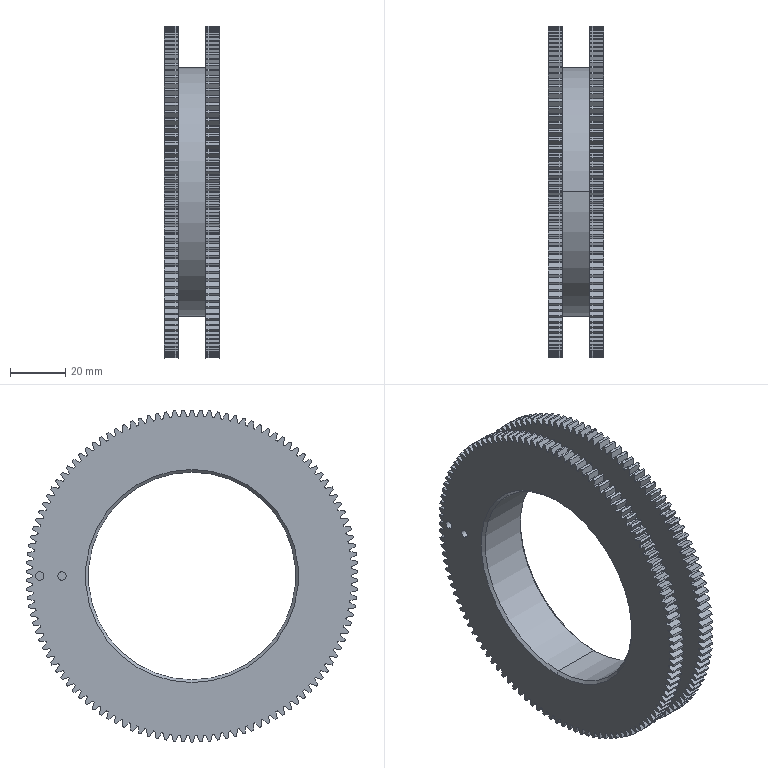Component | SolidWorks | 20Gear-2 | 1 solid | 962 faces | volume 84122 mm3 | cylinder 482 | plane 476 | cone 4 | commonest cylinder face diameters 120 x238 115.5 x236 3 x4 90 x2 75 x2